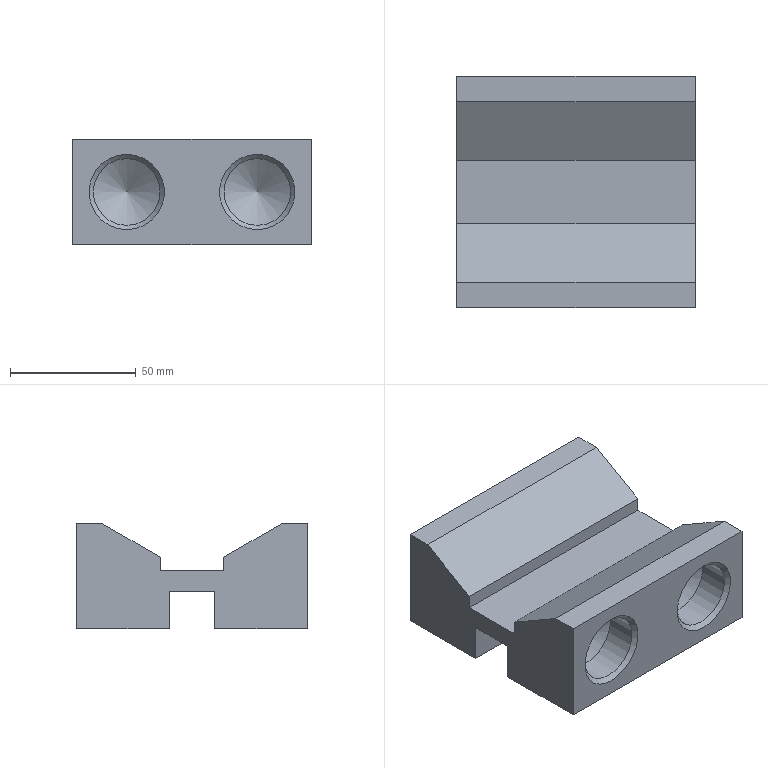Component | NX | BRACKET | 1 solid | 38 faces | volume 224336 mm3 | plane 18 | cone 12 | cylinder 8 | commonest cylinder face diameters 26.59 x4 8.5 x2 10 x2